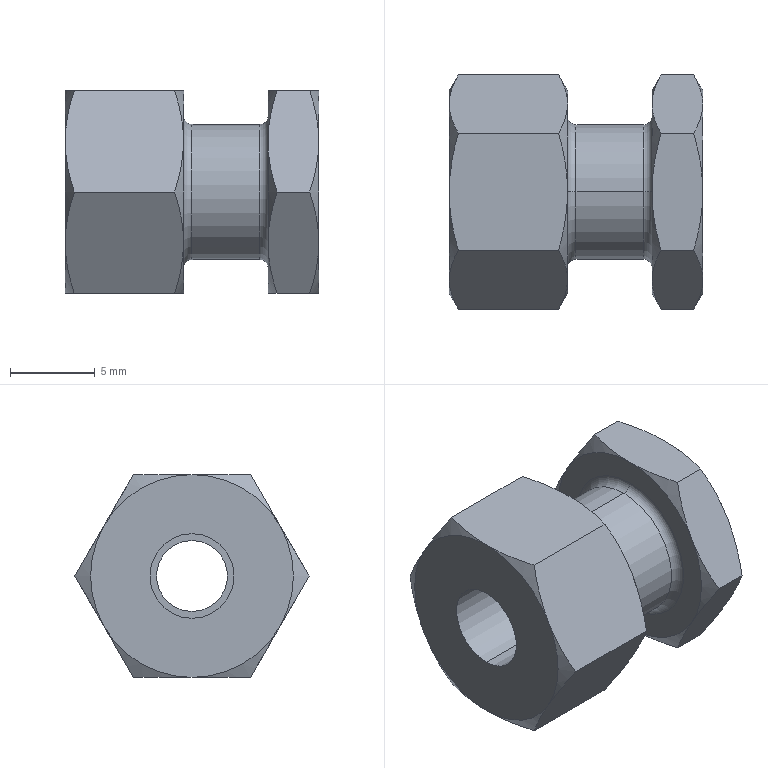Component | SolidWorks | 1BaseModel20210701145954-1 | 1 solid | 51 faces | volume 1240 mm3 | cone 24 | plane 17 | cylinder 6 | torus 4 | commonest cylinder face diameters 5 x2 8 x2 4.2 x2 | material Equivalent to S45C